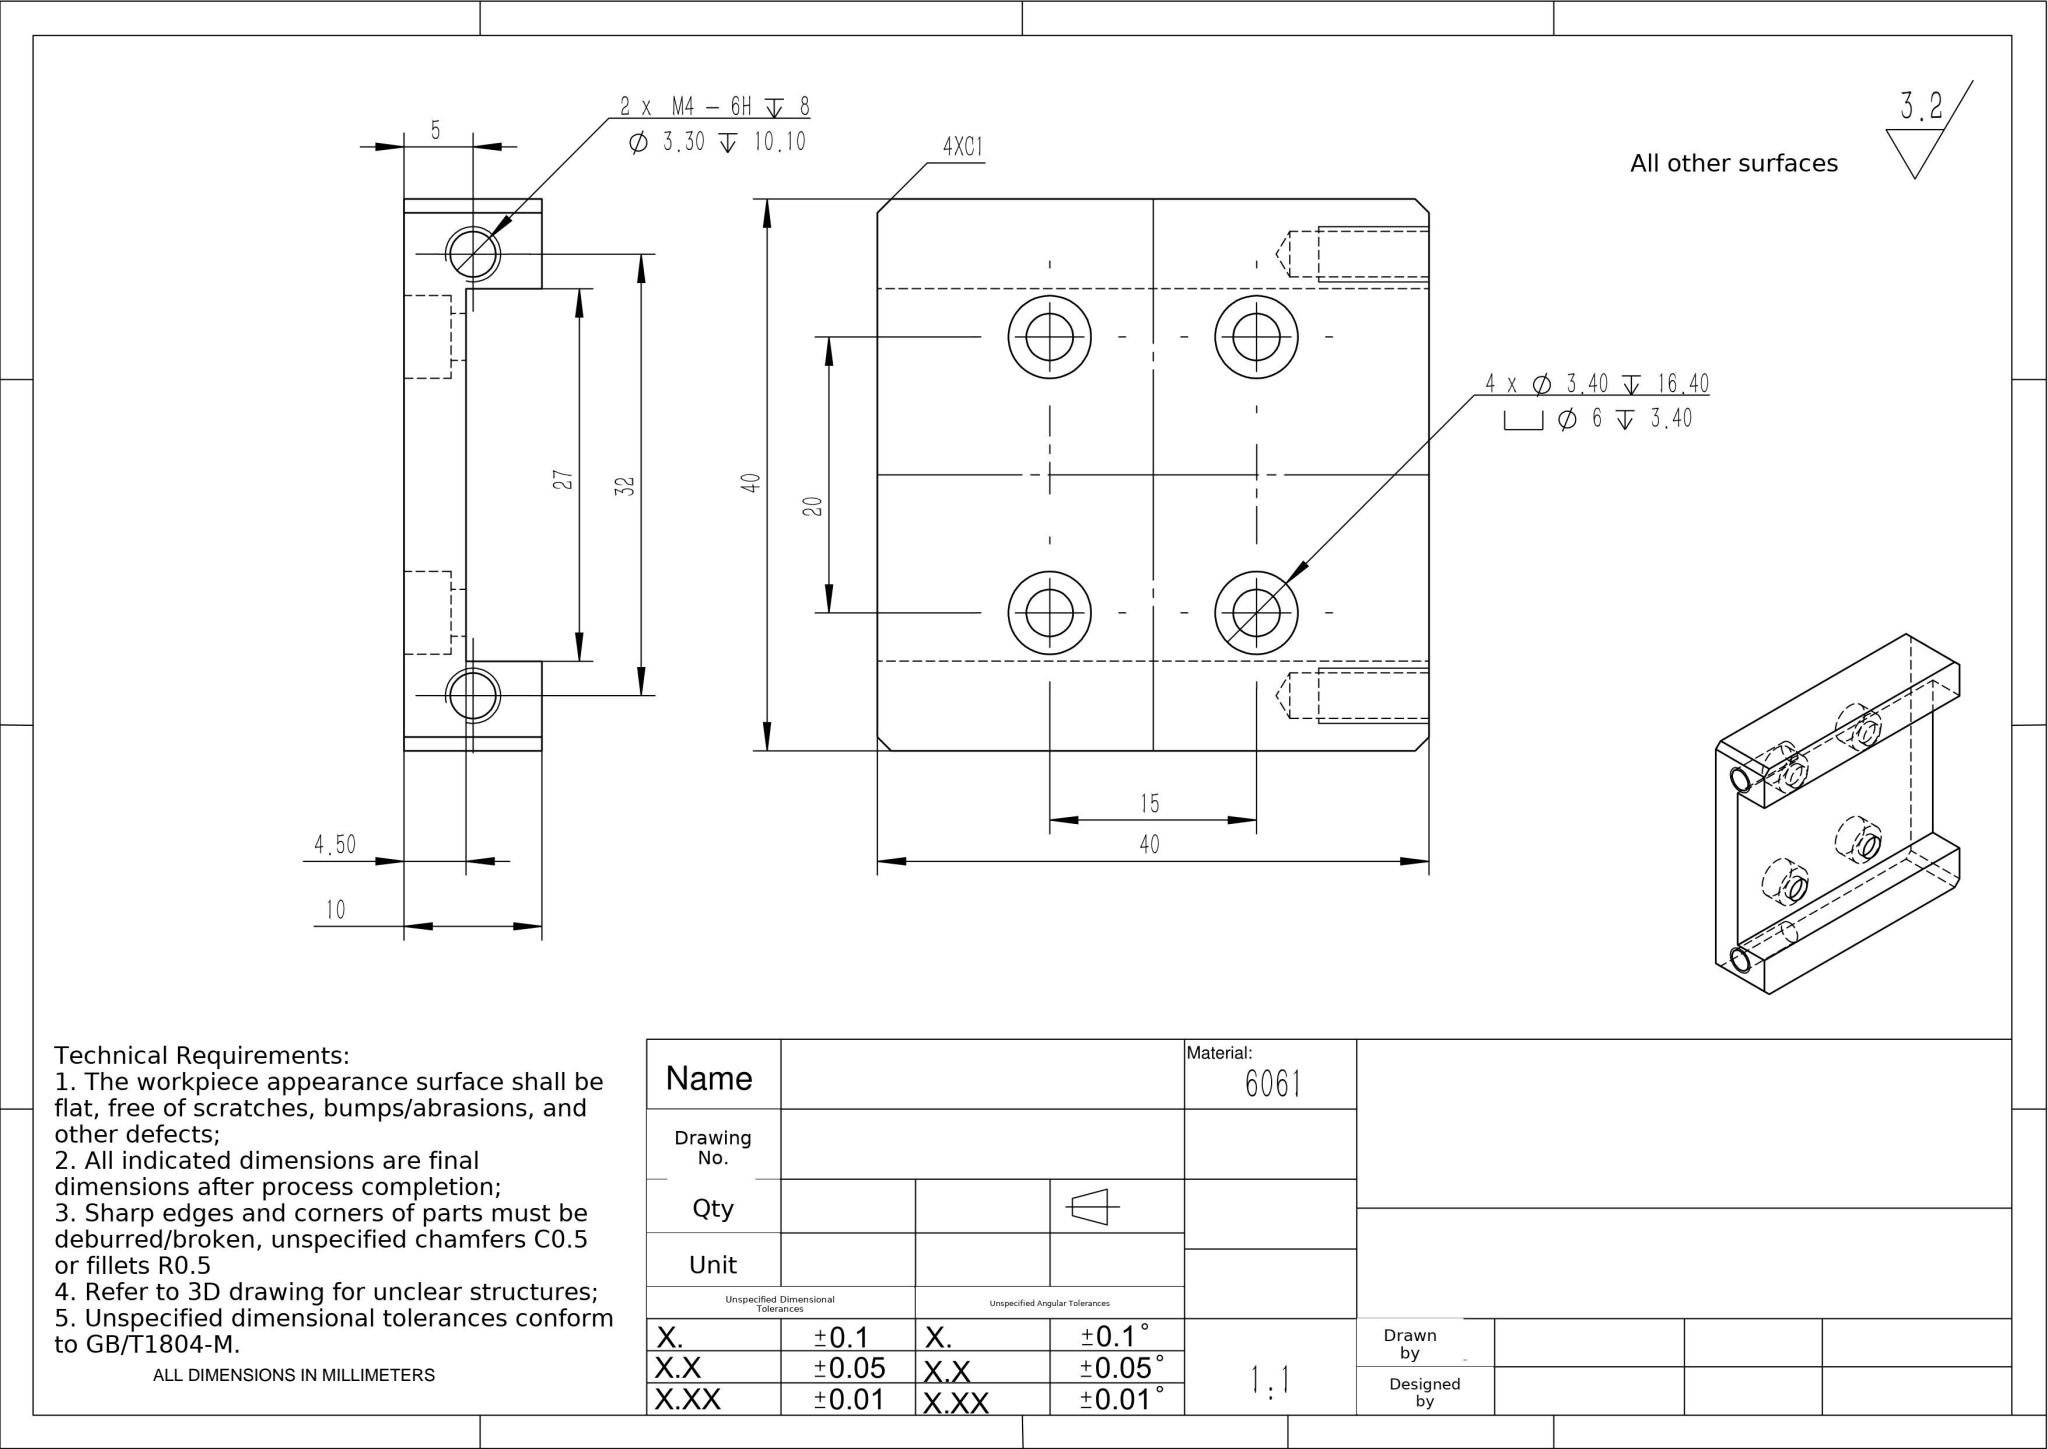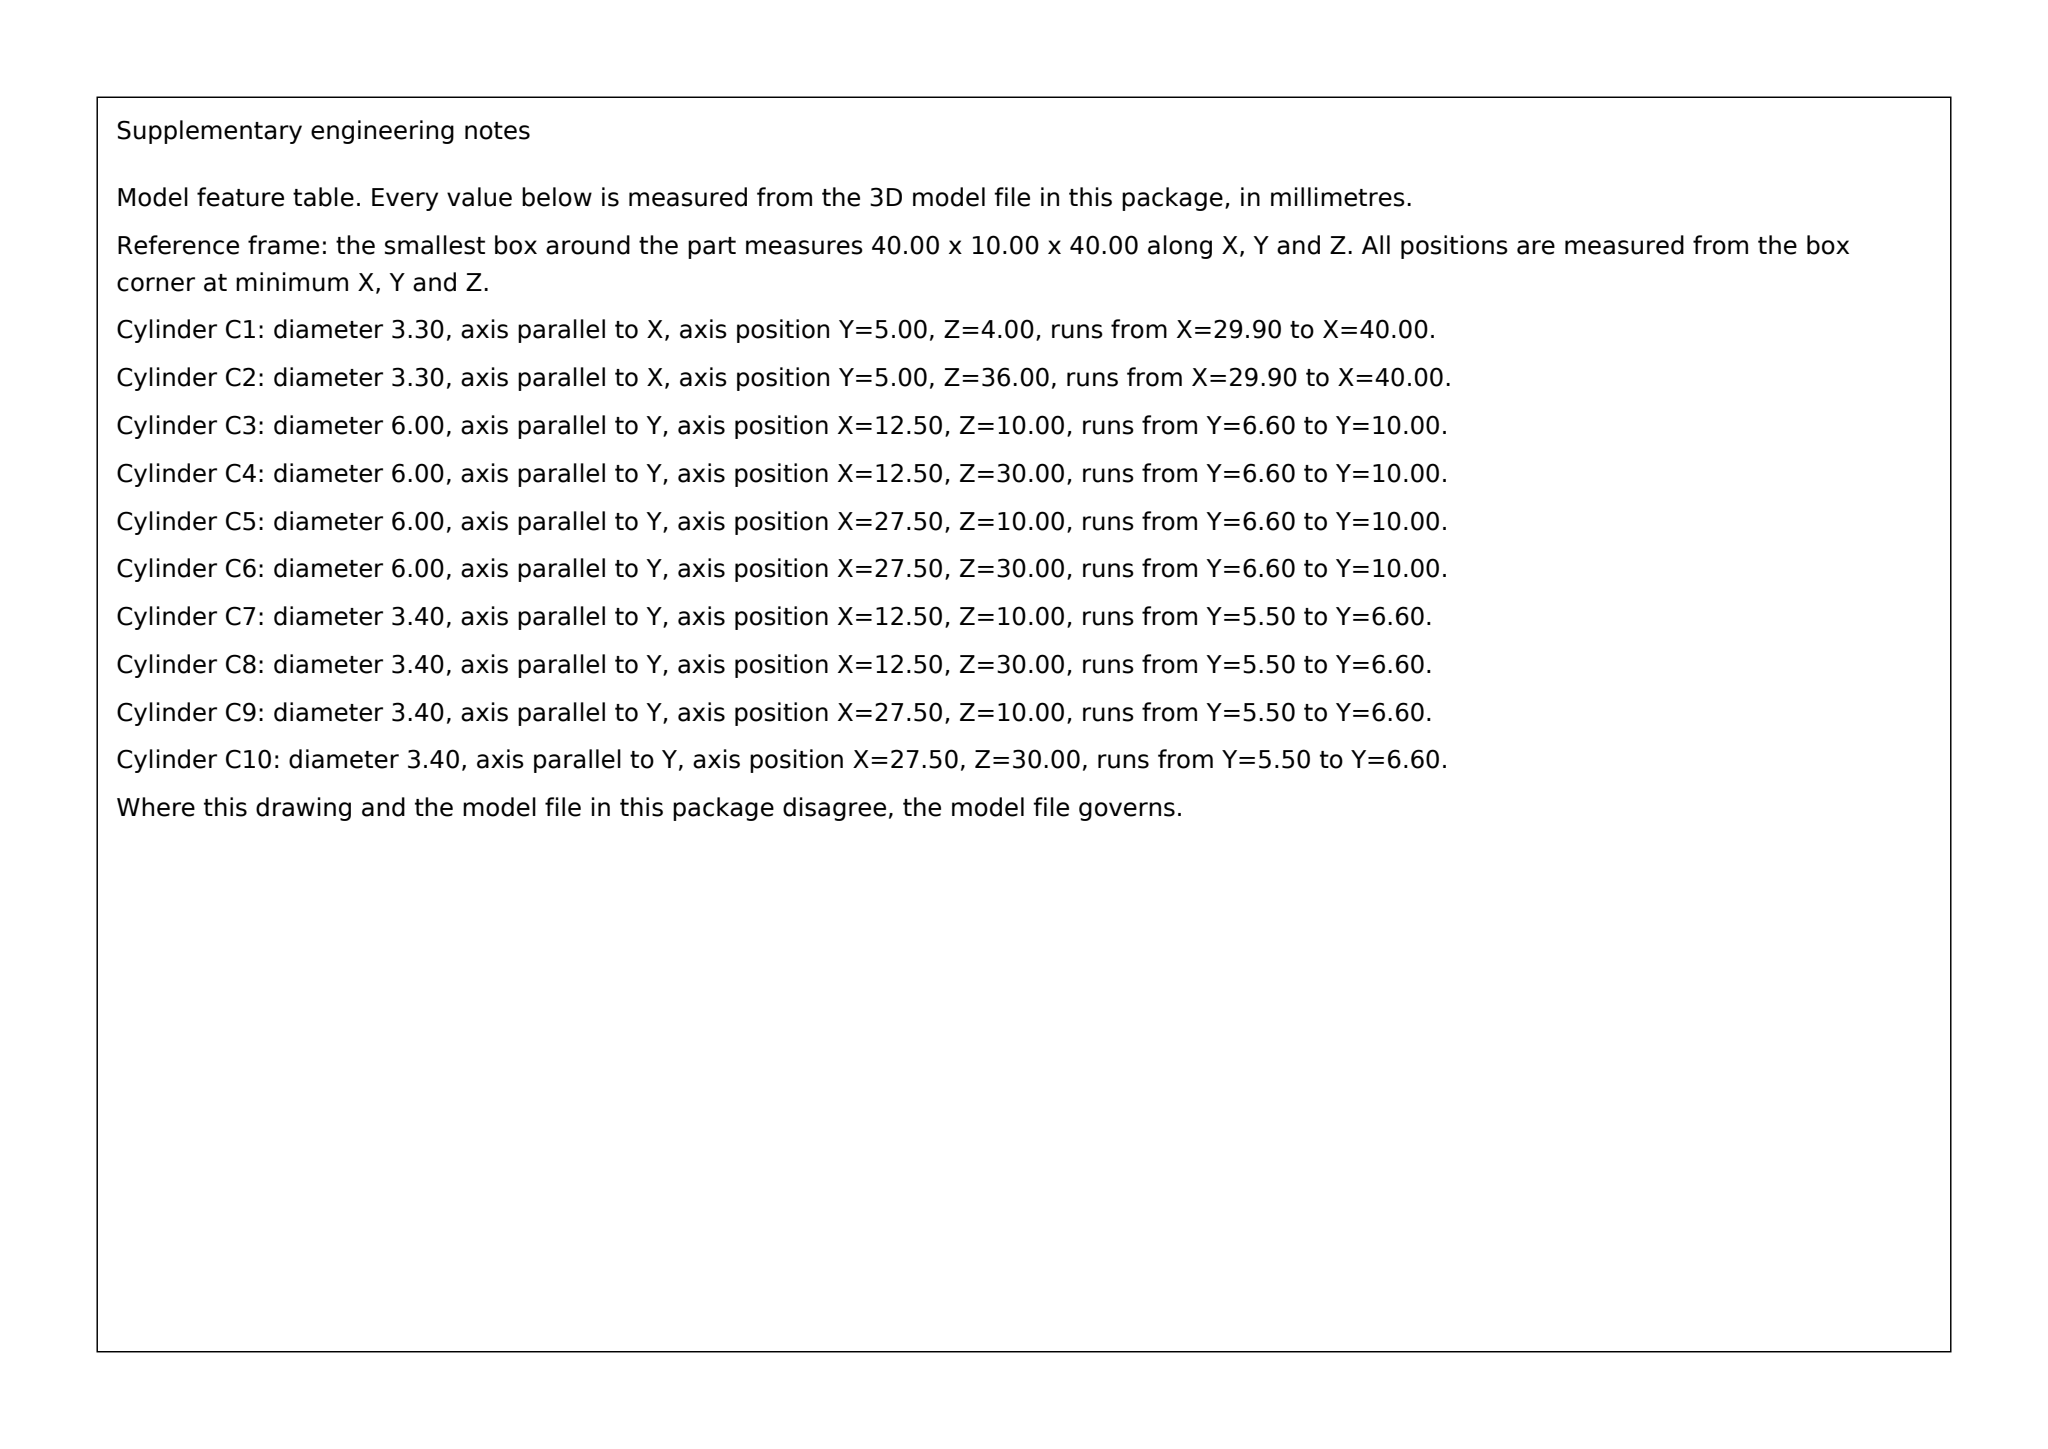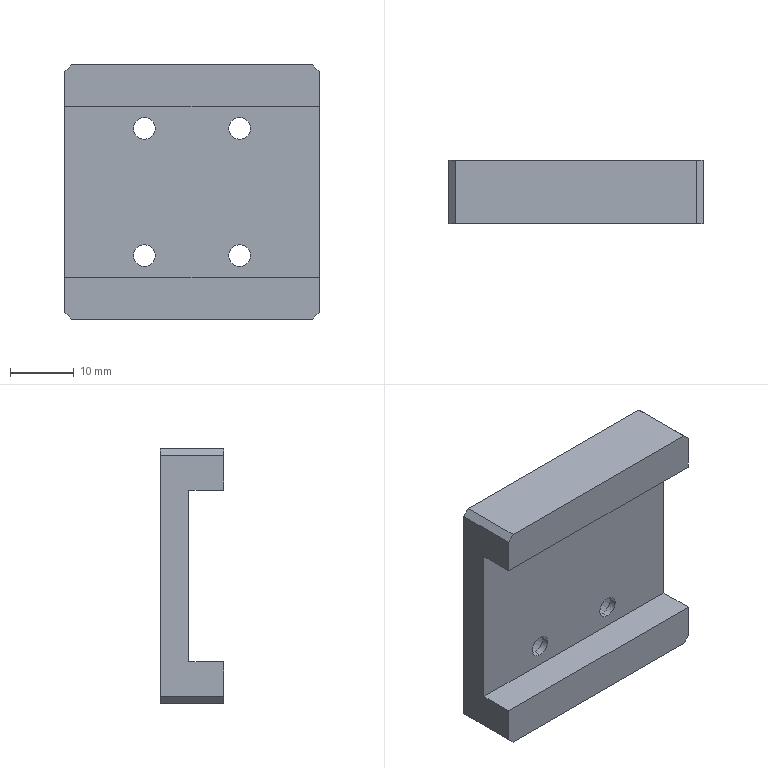Part | SolidWorks | mm | 1 solid | 42 faces | box 40 x 10 x 40 mm | volume 9437 mm3 | cylinder 20 | plane 18 | cone 4 | commonest cylinder face diameters 6 x8 3.4 x8 3.3 x4
build123d program:
from build123d import *

# Parameters (mm, degrees)
SKETCH1_W                                         = 40
SKETCH1_H                                         = 40
BOSS_EXTRUDE1_DEPTH                               = 10
SKETCH2_W                                         = 40
SKETCH2_H                                         = 27
CUT_EXTRUDE1_DEPTH                                = 5.5
HOLE_SIZE_ACCORDING_TO_TYPE_1_OF_HEXA_D           = 3.4
HOLE_SIZE_ACCORDING_TO_TYPE_1_OF_HEXA_DEPTH       = 16.4
HOLE_SIZE_ACCORDING_TO_TYPE_1_OF_HEXA_CBORE_D     = 6
HOLE_SIZE_ACCORDING_TO_TYPE_1_OF_HEXA_CBORE_DEPTH = 3.4
HOLE_SIZE_ACCORDING_TO_TYPE_1_OF_HEXA_TIP         = 1.021
M4_TAPPED_HOLE1_D                                 = 3.3
M4_TAPPED_HOLE1_DEPTH                             = 10.1
M4_TAPPED_HOLE1_TIP                               = 0.9914
CHAMFER1_SIZE                                     = 1


with BuildPart() as part:
    # Sketch1 → Boss-Extrude1 (new body)
    with BuildSketch(Plane(origin=(0, 0, 0), x_dir=(1, 0, 0), z_dir=(0, 1, 0))):
        Rectangle(SKETCH1_W, SKETCH1_H)
    extrude(amount=BOSS_EXTRUDE1_DEPTH)

    # Sketch2 → Cut-Extrude1 (cut)
    with BuildSketch(Plane.XZ):
        Rectangle(SKETCH2_W, SKETCH2_H)
    extrude(amount=-CUT_EXTRUDE1_DEPTH, mode=Mode.SUBTRACT)

    # Hole Size _ according to_ Type 1 of Hexa
    with Locations(Plane(origin=(-7.5, 10, -10), x_dir=(0, 0, 1), z_dir=(0, 1, 0))):
        with Locations((0, 0), (0, 15), (20, 15), (20, 0)):
            CounterBoreHole(HOLE_SIZE_ACCORDING_TO_TYPE_1_OF_HEXA_D / 2, HOLE_SIZE_ACCORDING_TO_TYPE_1_OF_HEXA_CBORE_D / 2, HOLE_SIZE_ACCORDING_TO_TYPE_1_OF_HEXA_CBORE_DEPTH, depth=HOLE_SIZE_ACCORDING_TO_TYPE_1_OF_HEXA_DEPTH)
            with Locations((0, 0, -(HOLE_SIZE_ACCORDING_TO_TYPE_1_OF_HEXA_DEPTH + HOLE_SIZE_ACCORDING_TO_TYPE_1_OF_HEXA_TIP / 2))):  # 118° drill point
                Cone(0, HOLE_SIZE_ACCORDING_TO_TYPE_1_OF_HEXA_D / 2, HOLE_SIZE_ACCORDING_TO_TYPE_1_OF_HEXA_TIP, mode=Mode.SUBTRACT)

    # M4 Tapped Hole1
    with Locations(Plane(origin=(20, 5, 16), x_dir=(0, 0, 1), z_dir=(1, 0, 0))):
        with Locations((0, 0), (-32, 0)):
            Hole(M4_TAPPED_HOLE1_D / 2, depth=M4_TAPPED_HOLE1_DEPTH)
            with Locations((0, 0, -(M4_TAPPED_HOLE1_DEPTH + M4_TAPPED_HOLE1_TIP / 2))):  # 118° drill point
                Cone(0, M4_TAPPED_HOLE1_D / 2, M4_TAPPED_HOLE1_TIP, mode=Mode.SUBTRACT)

    # Chamfer1
    chamfer1_edges = [part.edges().sort_by_distance(p)[0] for p in [
        (20, 5, 20),
        (-20, 5, 20),
        (-20, 5, -20),
        (20, 5, -20),
    ]]
    chamfer(chamfer1_edges, length=CHAMFER1_SIZE)


solid = part.part